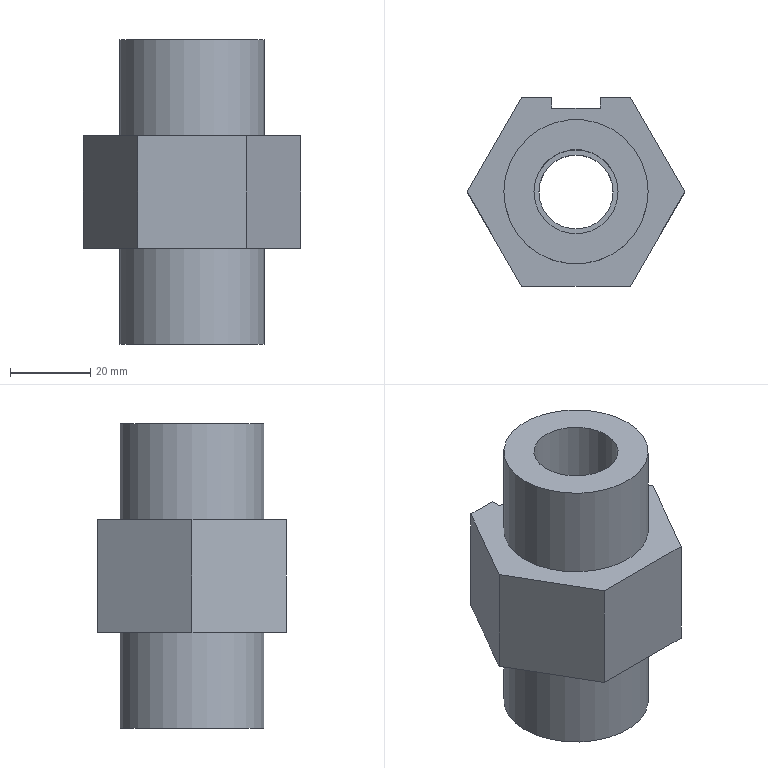CAM job | NX | mm | 3+2-indexed | 1 set-up | 9 operations | part box 54.27 x 47 x 76
set-up 1
1. Planar Milling | Mill Mill5 T1 | PLANAR_PROFILE | path 13131.478 mm | 8.612 min
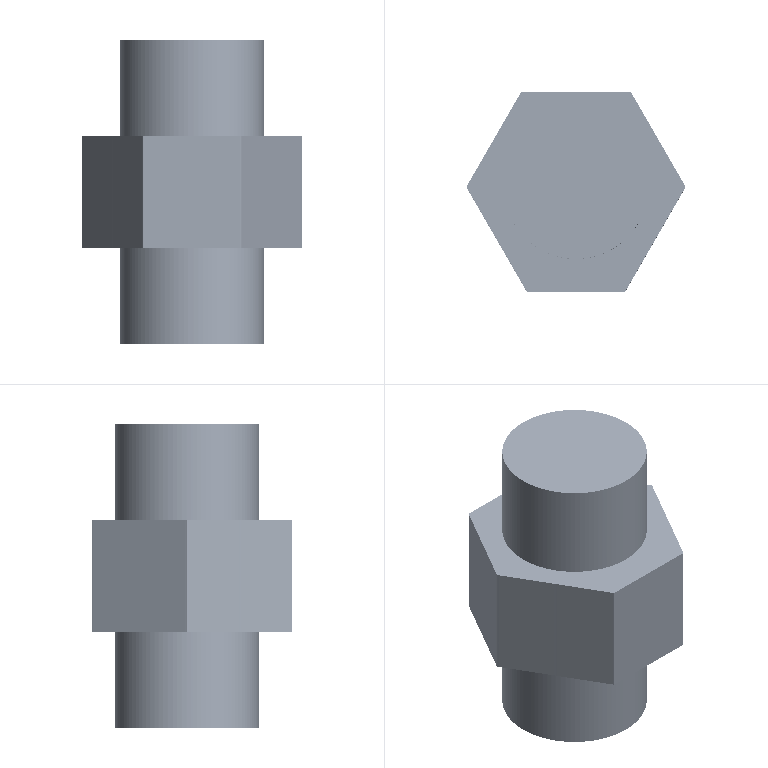2. Planar Milling | Mill Mill5 T2 | PLANAR_PROFILE_COPY | path 296.456 mm | 0.2752 min
3. Planar Milling | Mill Mill5 T3 | PLANAR_PROFILE_1 | path 760.579 mm | 0.4474 min
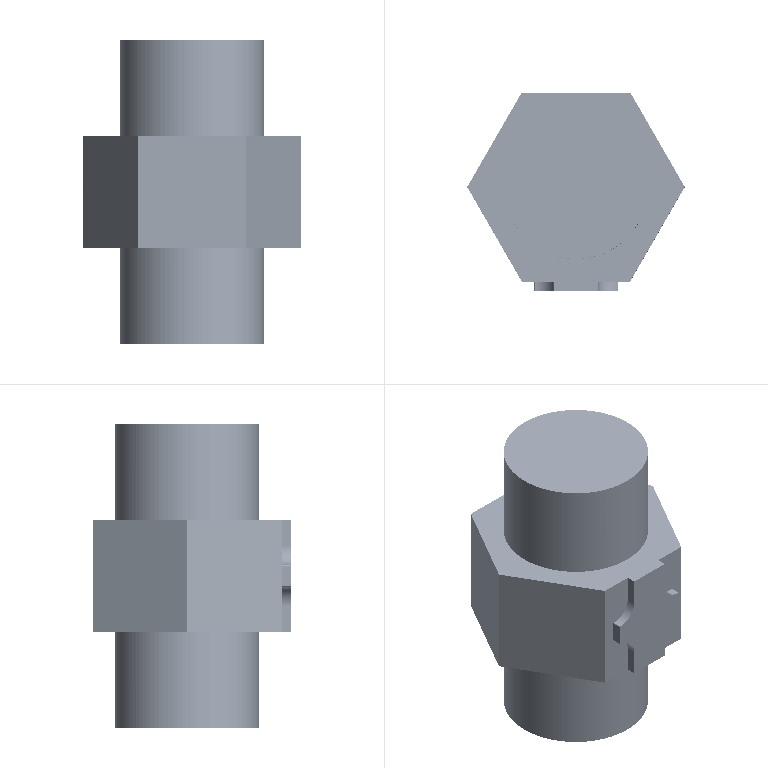4. Planar Milling | Mill Mill5 T4 | PLANAR_PROFILE_1_COPY | path 173.2 mm | 0.1342 min
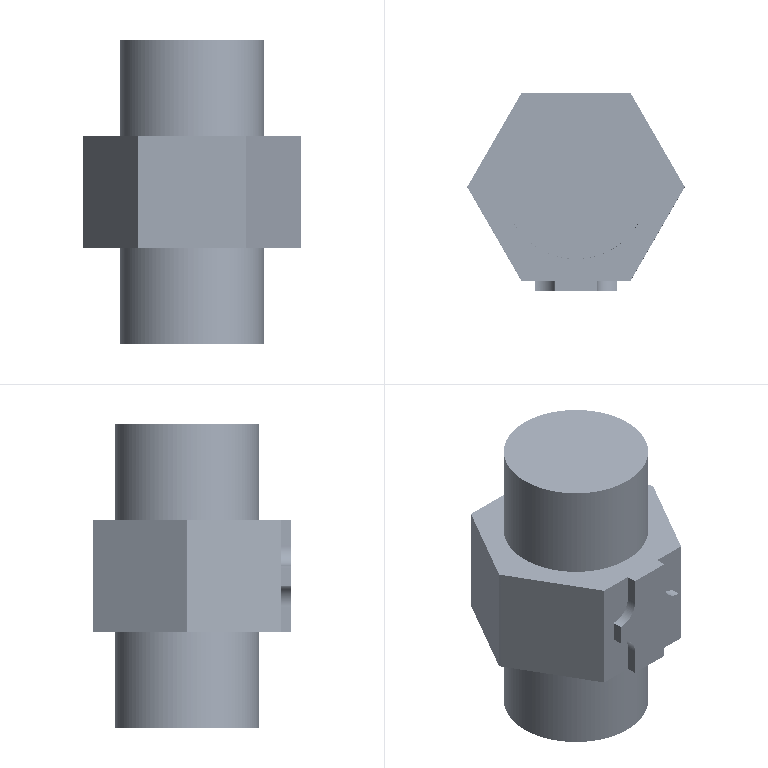5. Planar Milling | Mill Mill5 T5 | PLANAR_PROFILE_2 | path 261.911 mm | 0.1912 min
6. Planar Milling | Mill Mill5 T6 | PLANAR_PROFILE_3 | path 612.559 mm | 0.2148 min
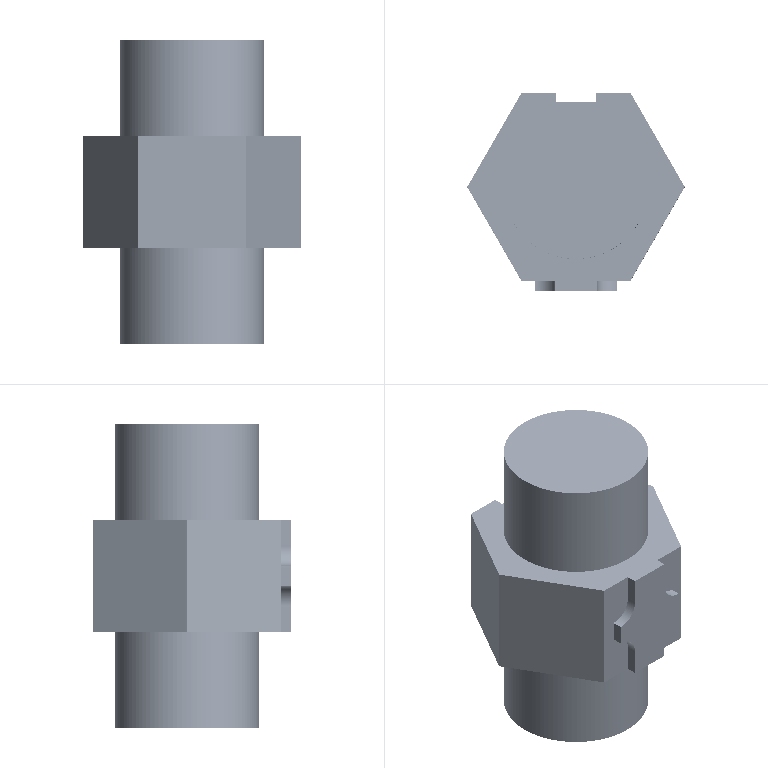7. Planar Milling | Mill Mill5 T7 | PLANAR_PROFILE_4 | path 77.895 mm | 0.05954 min
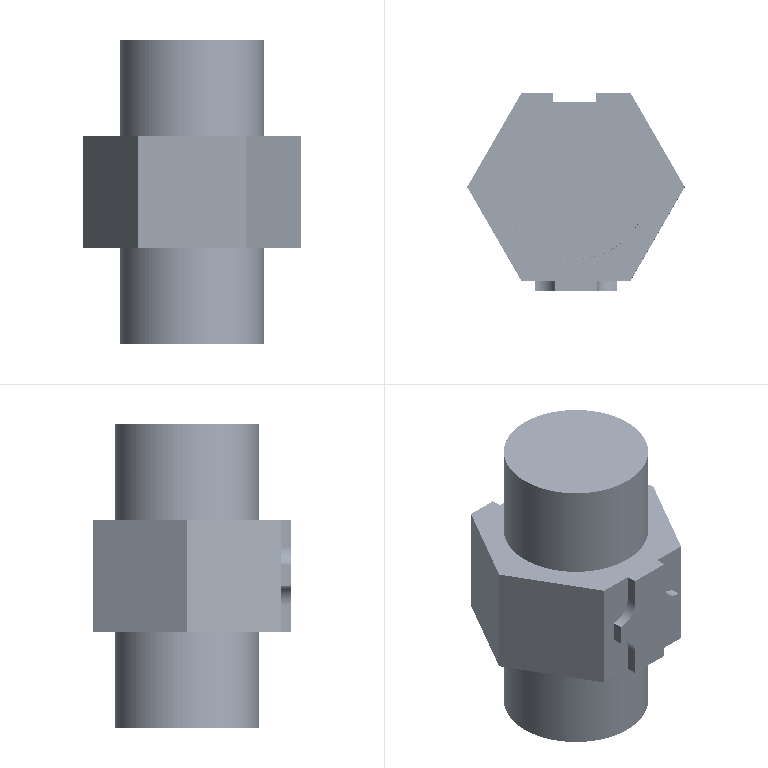8. Planar Milling | Mill Mill5 T8 | PLANAR_PROFILE_4_COPY | path 77.895 mm | 0.05954 min
9. Planar Milling | Mill Mill5 T9 | PLANAR_PROFILE_5 | path 172.272 mm | 0.1365 min